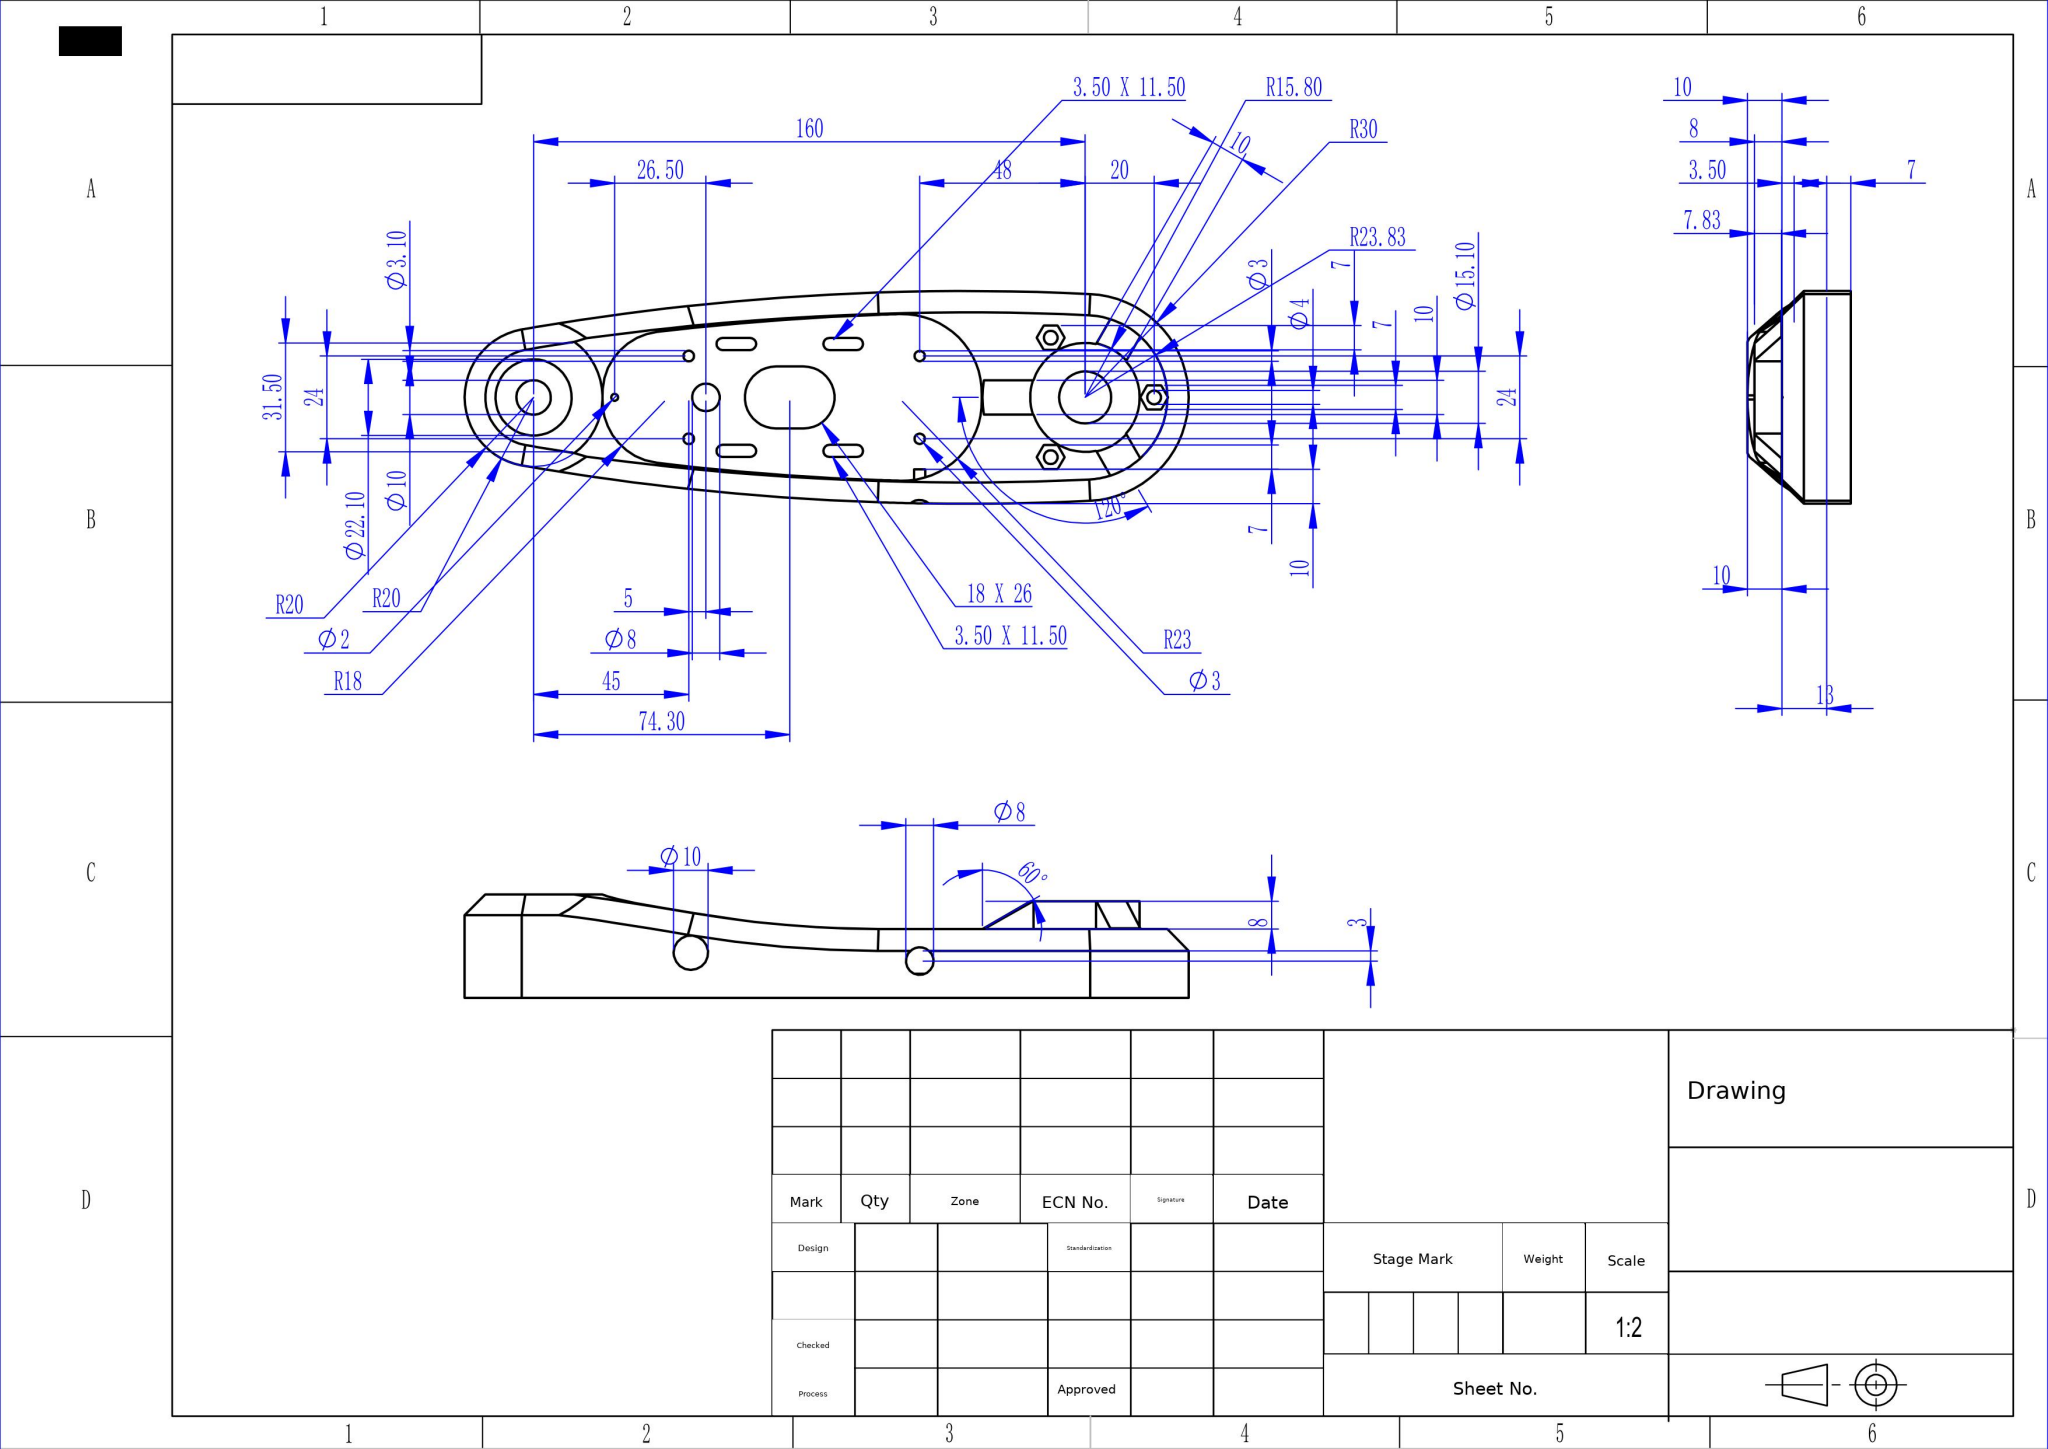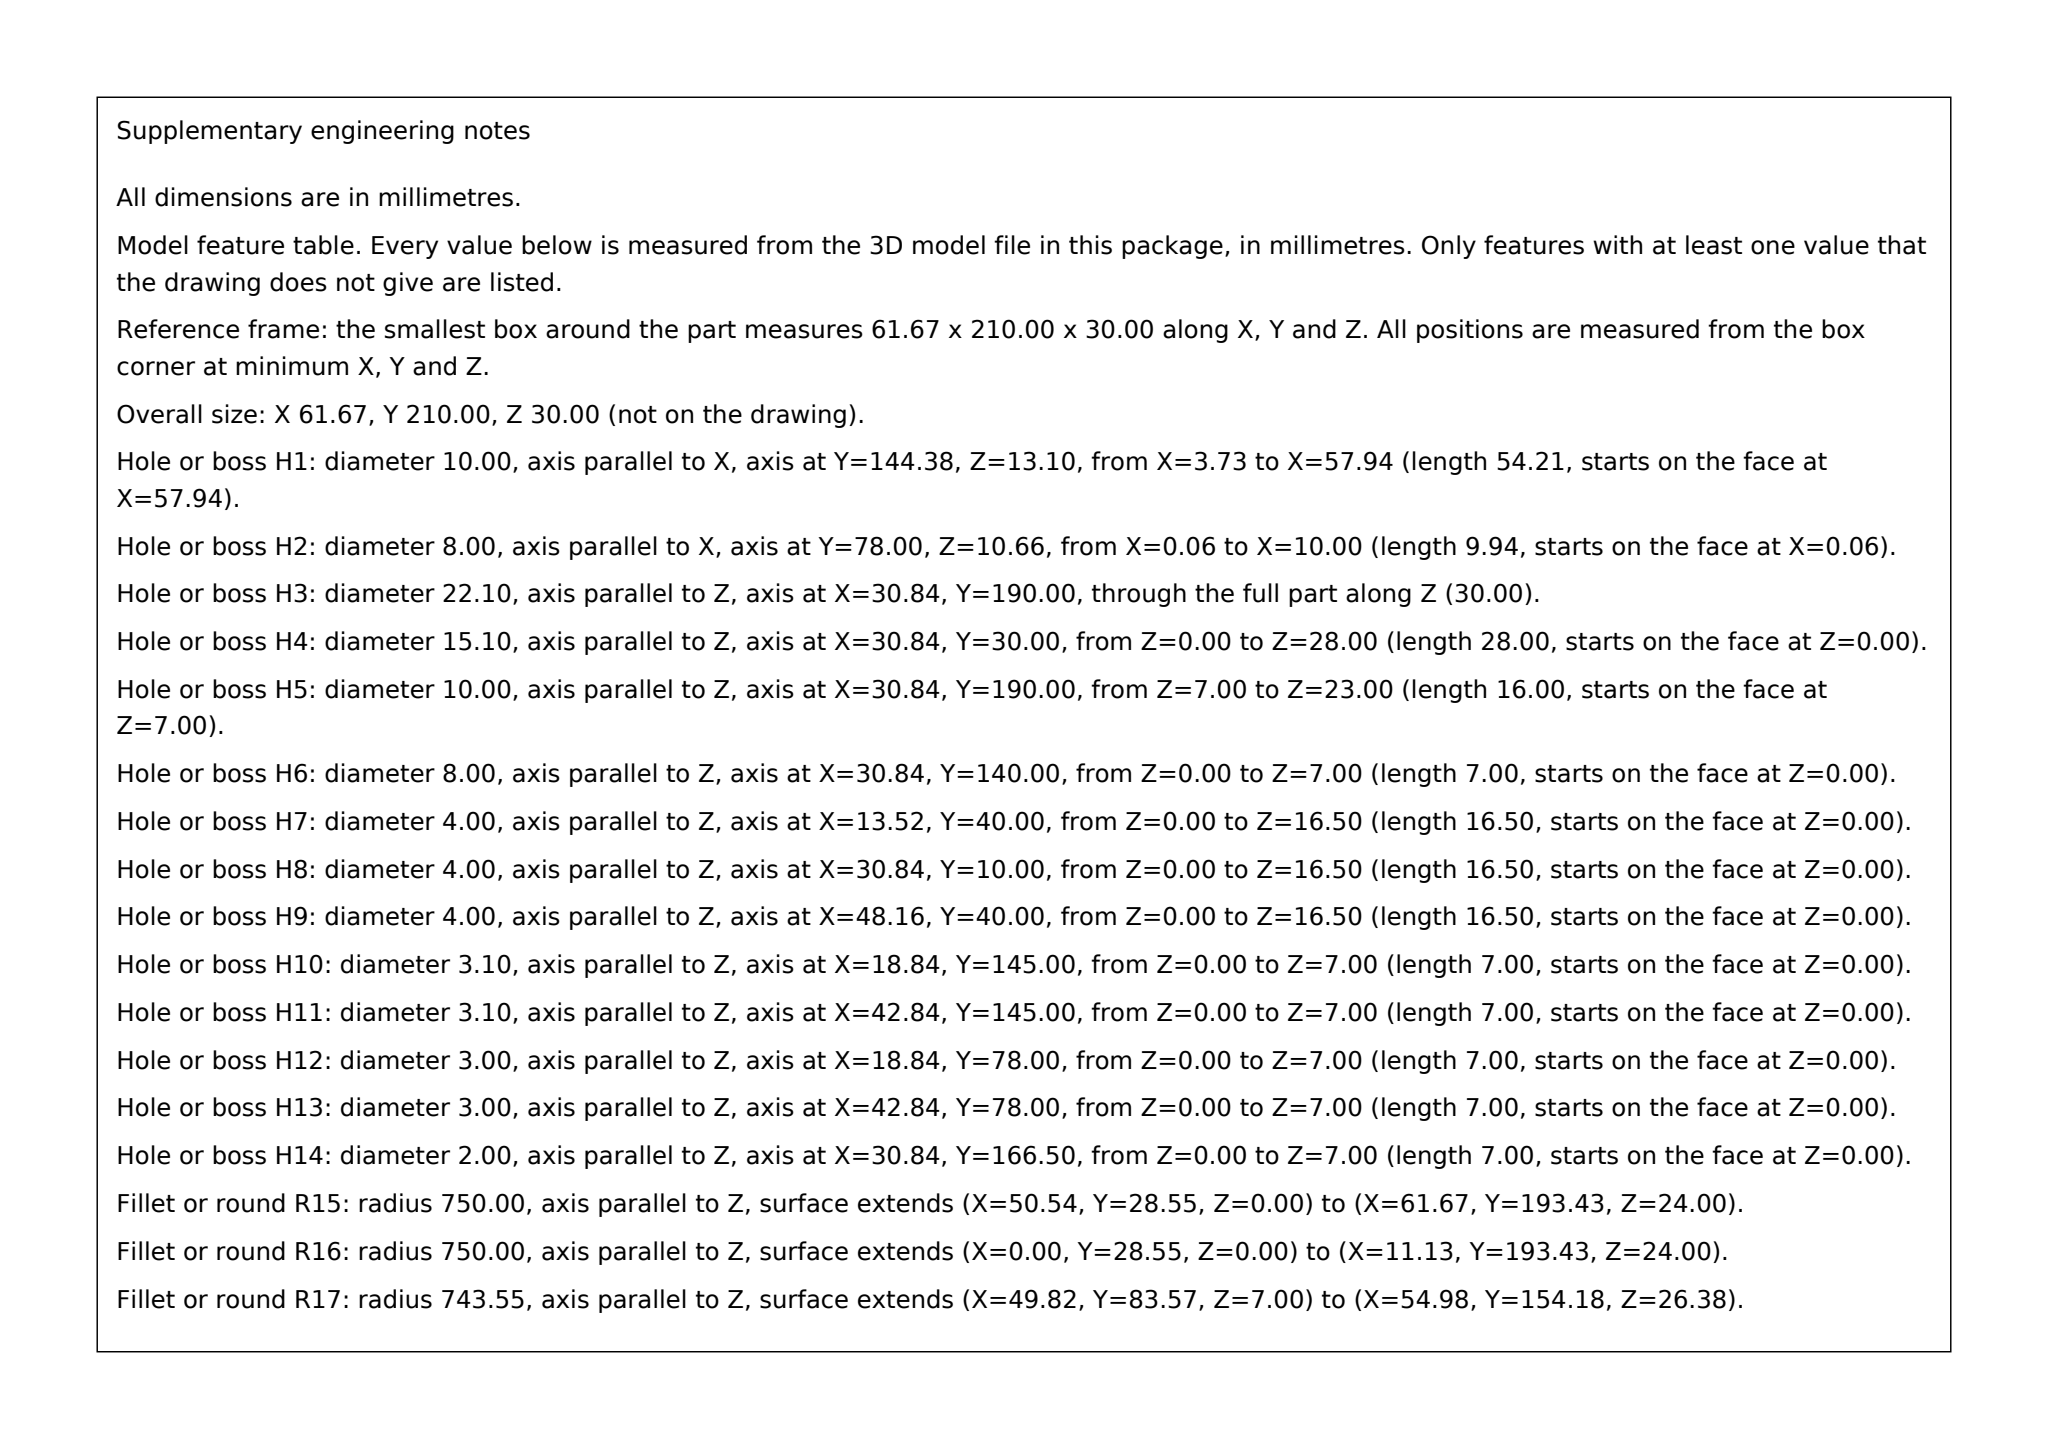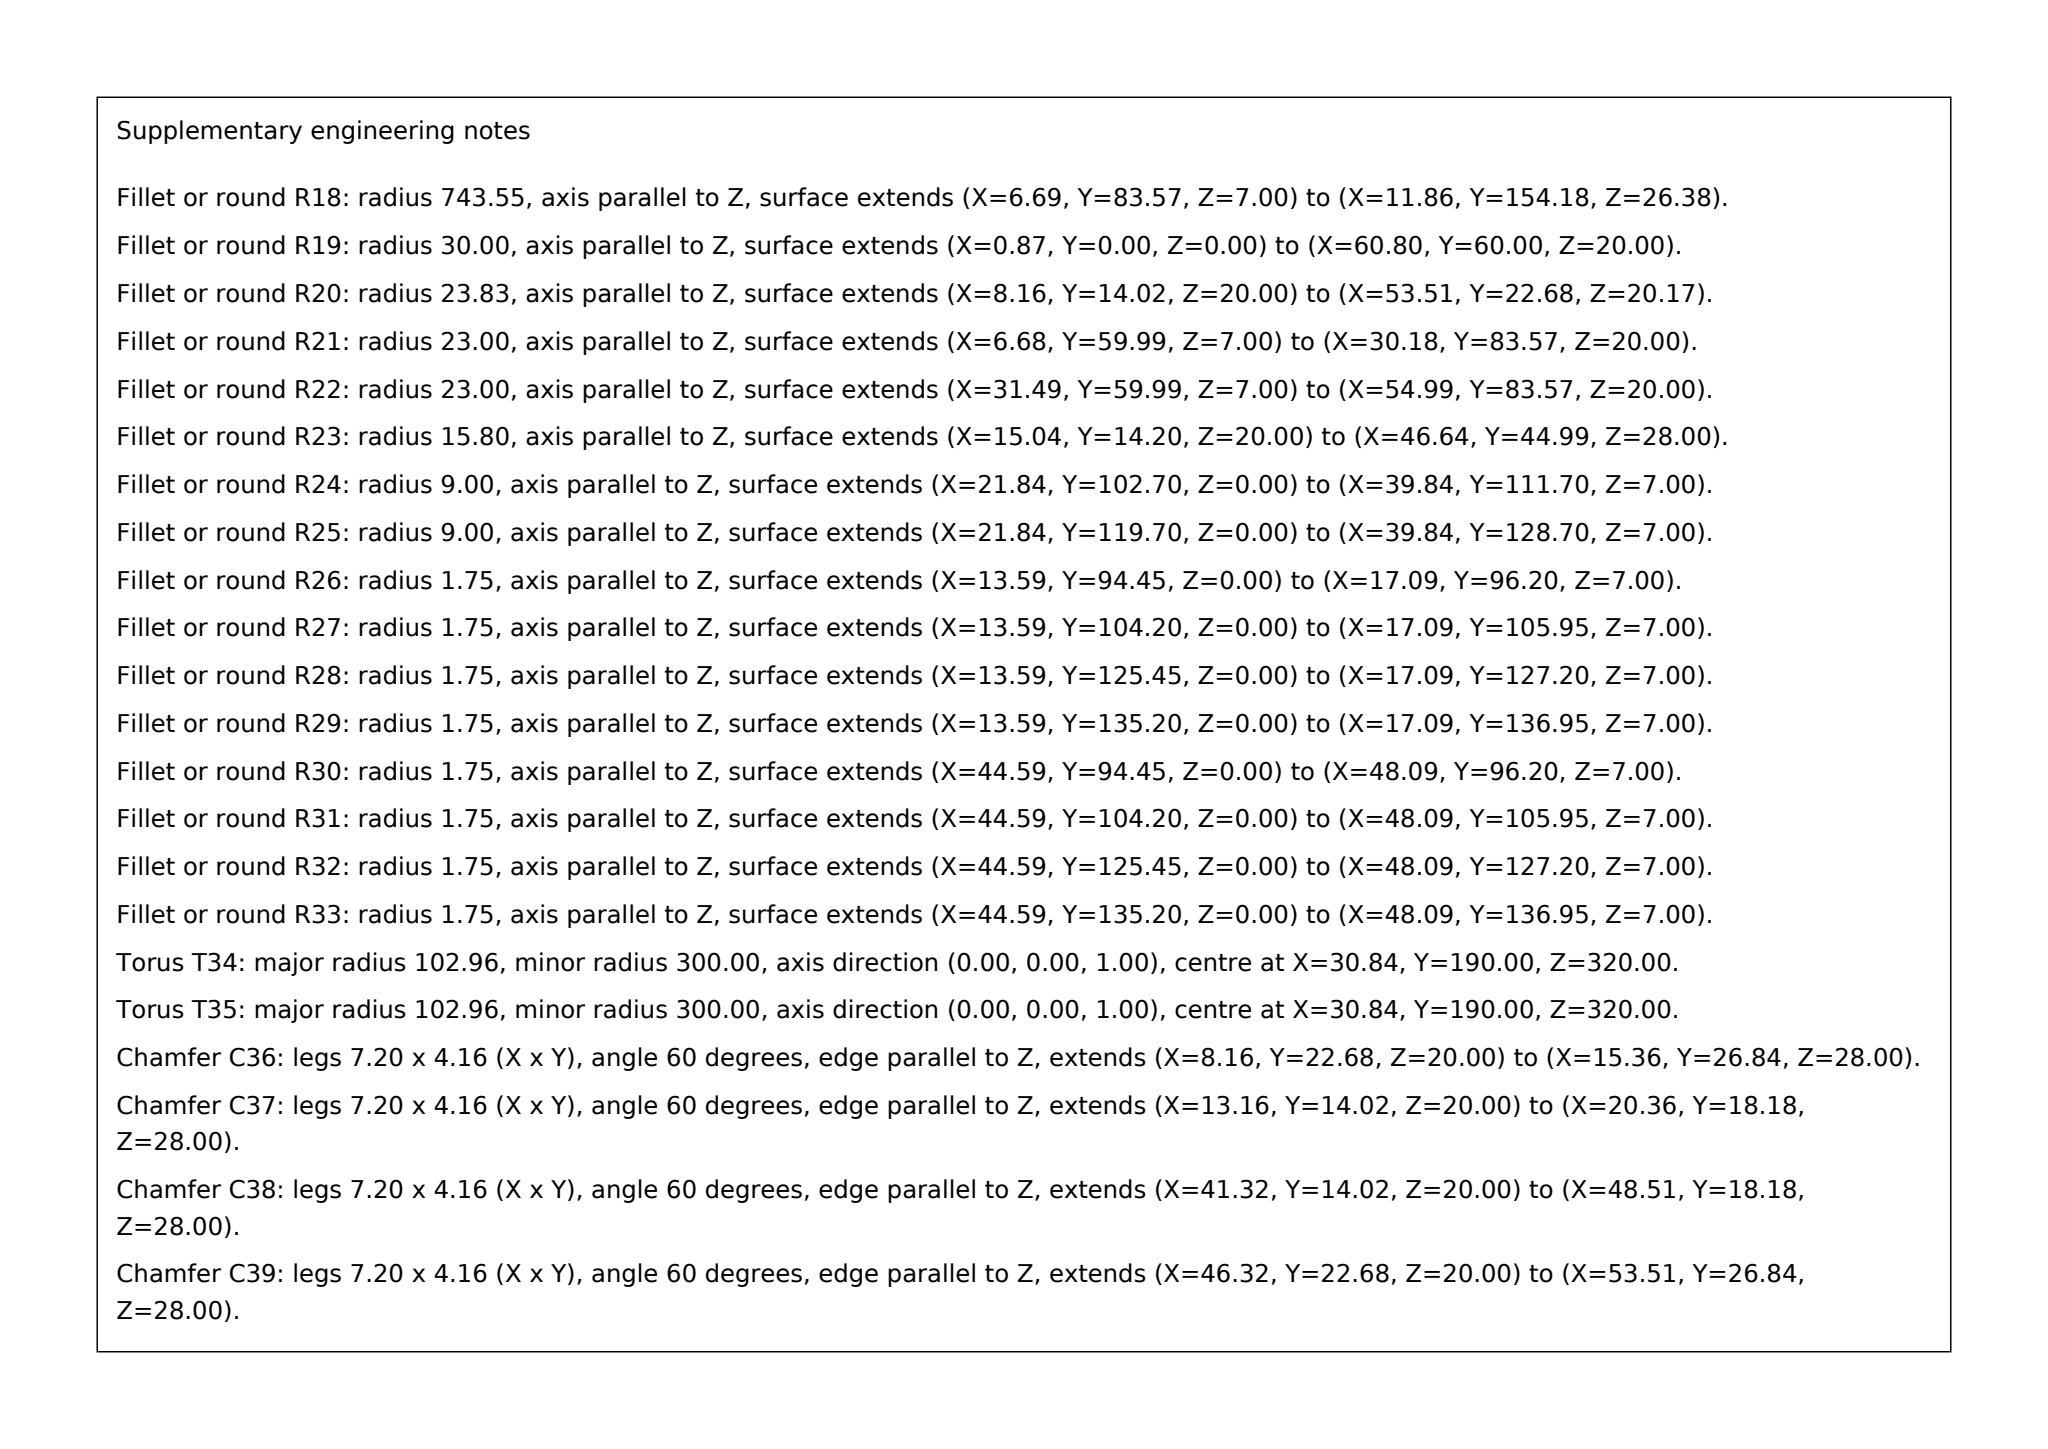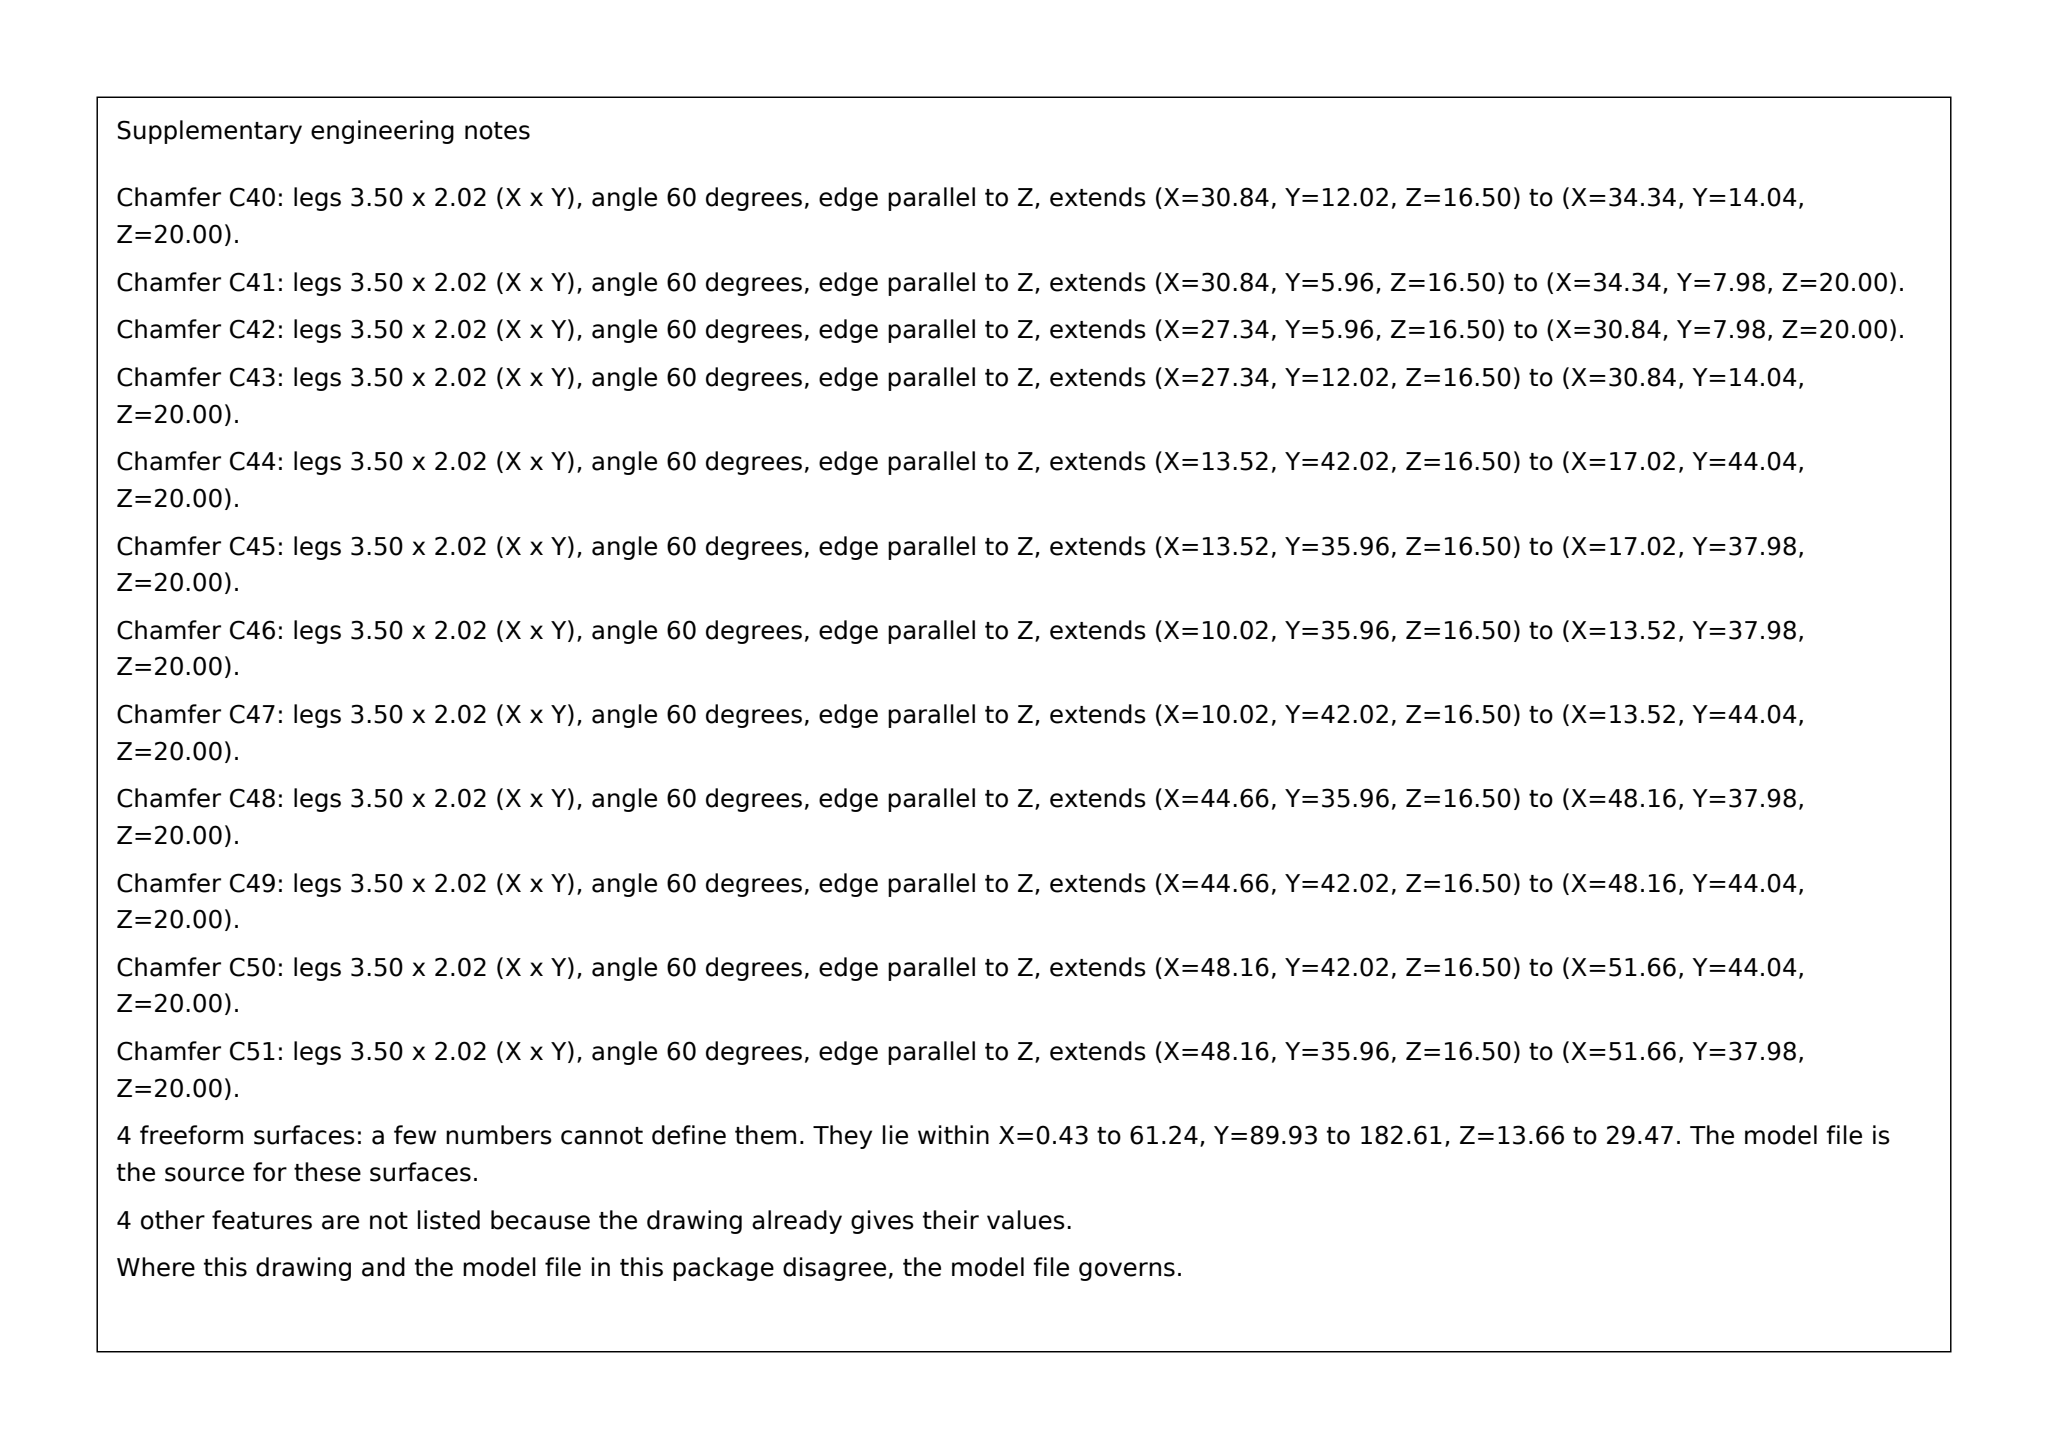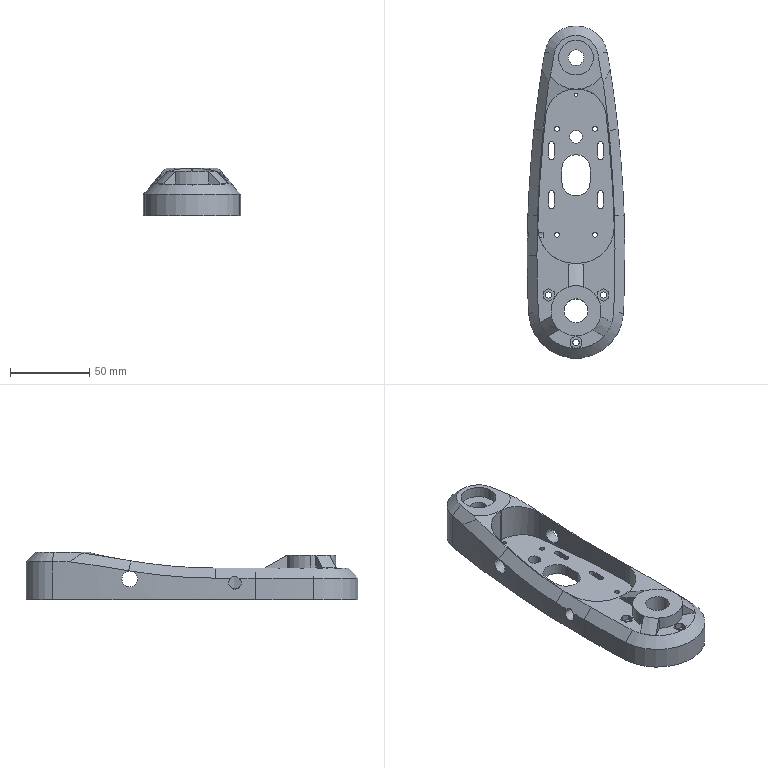Part | SolidWorks | mm | 1 solid | 129 faces | box 61.67 x 210 x 30 mm | volume 161077 mm3 | cylinder 64 | plane 47 | cone 12 | spline 4 | torus 2 | commonest cylinder face diameters 3.5 x8 10 x6 4 x6 2 x4 8 x4 31.6 x4 22.1 x4 3 x4